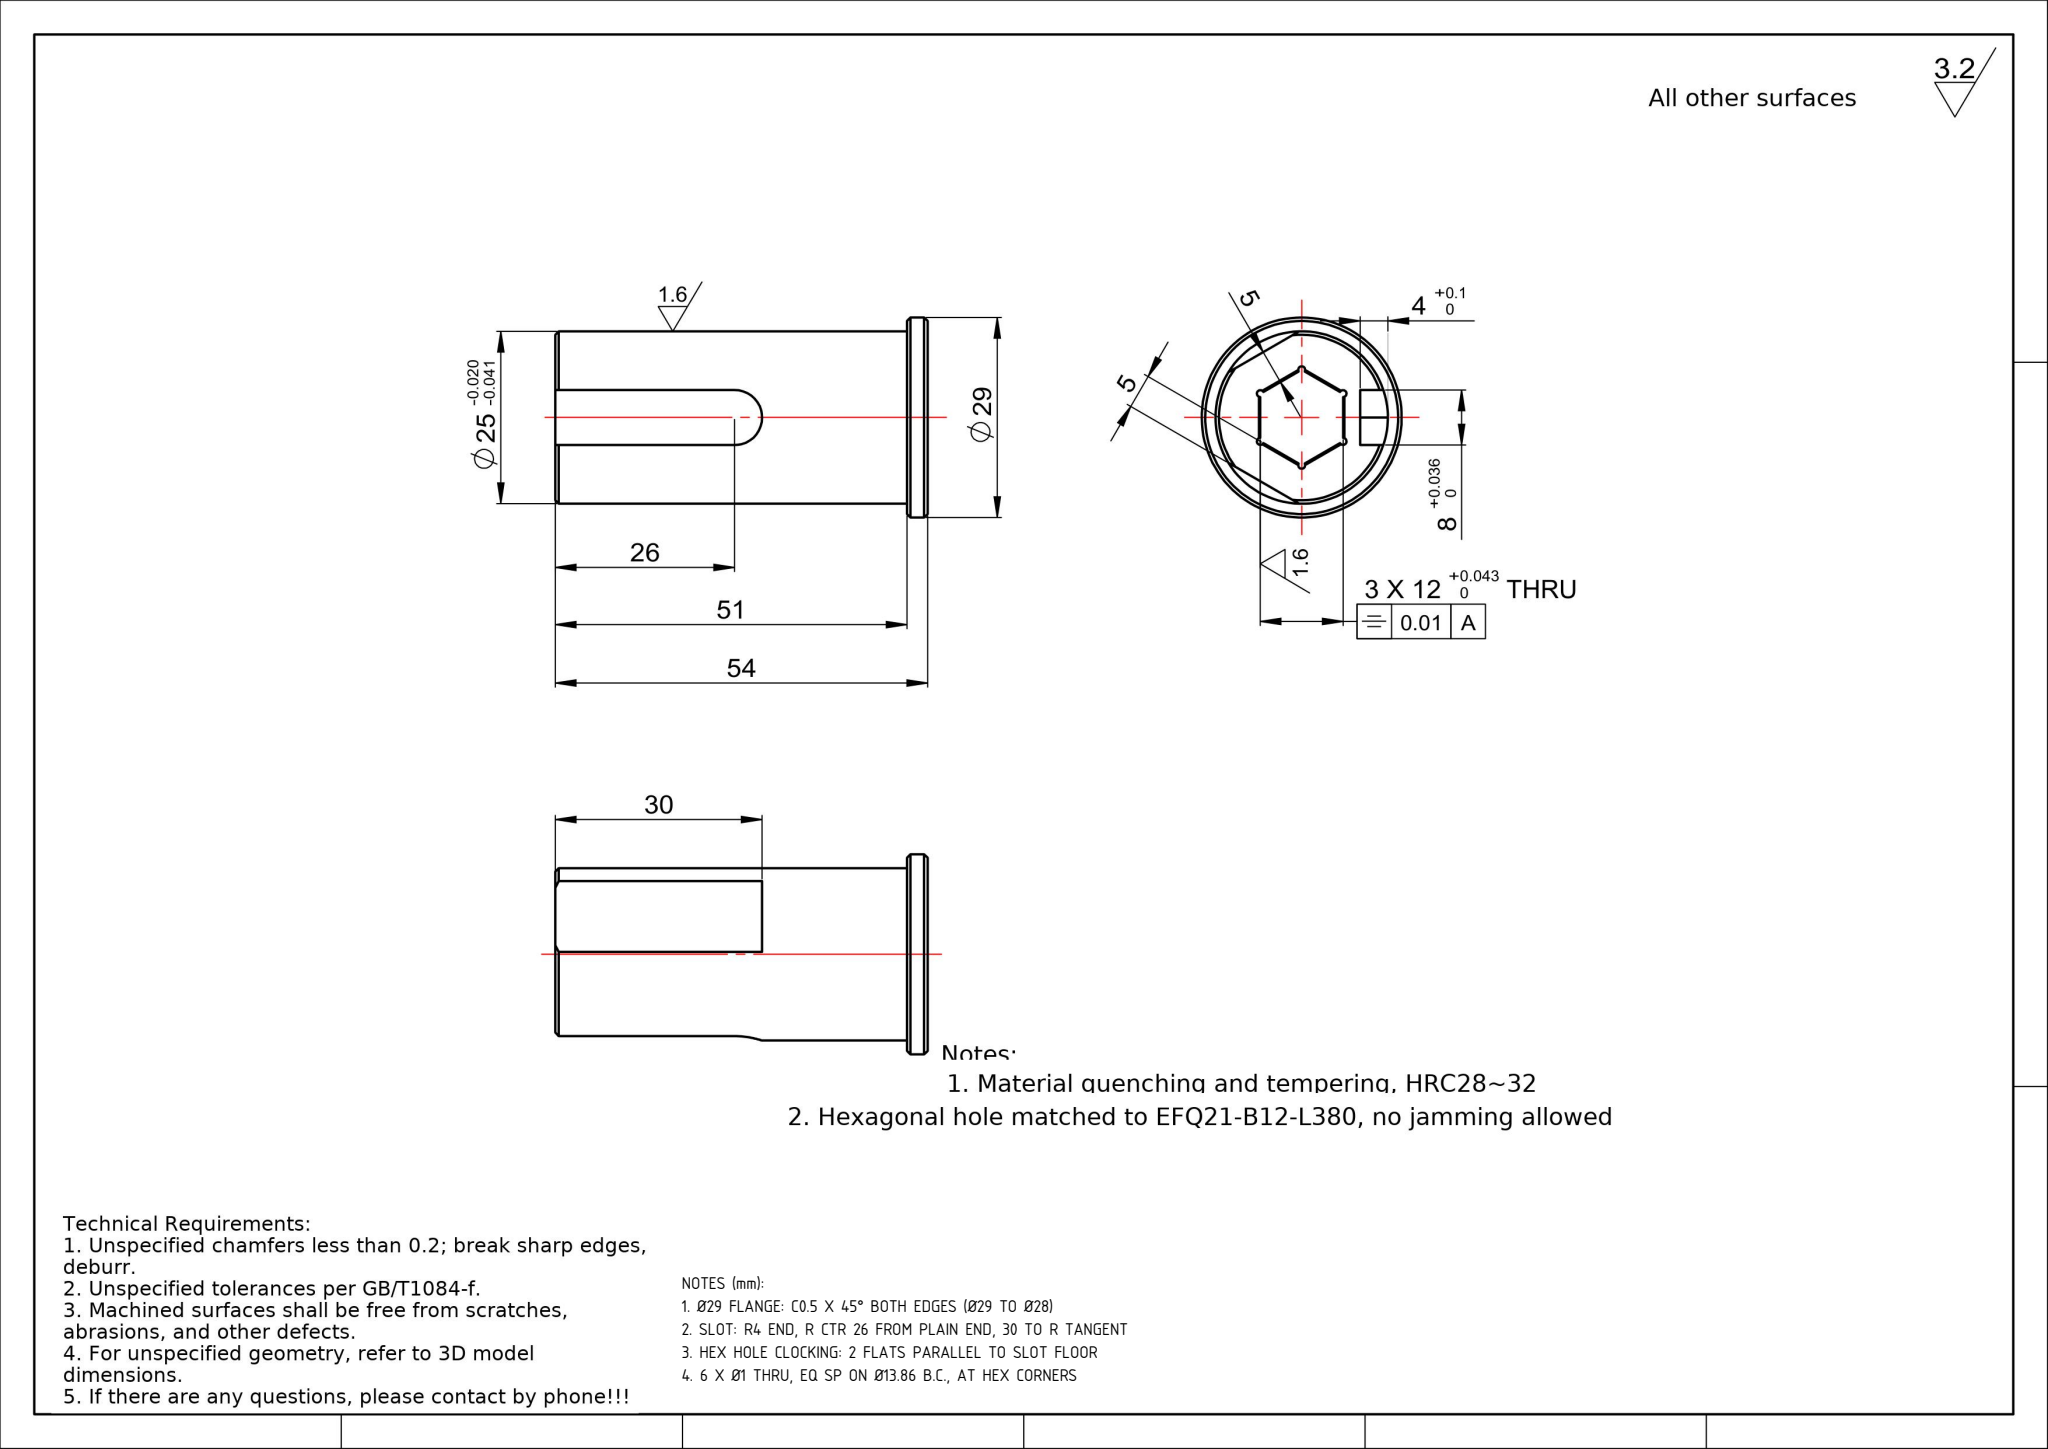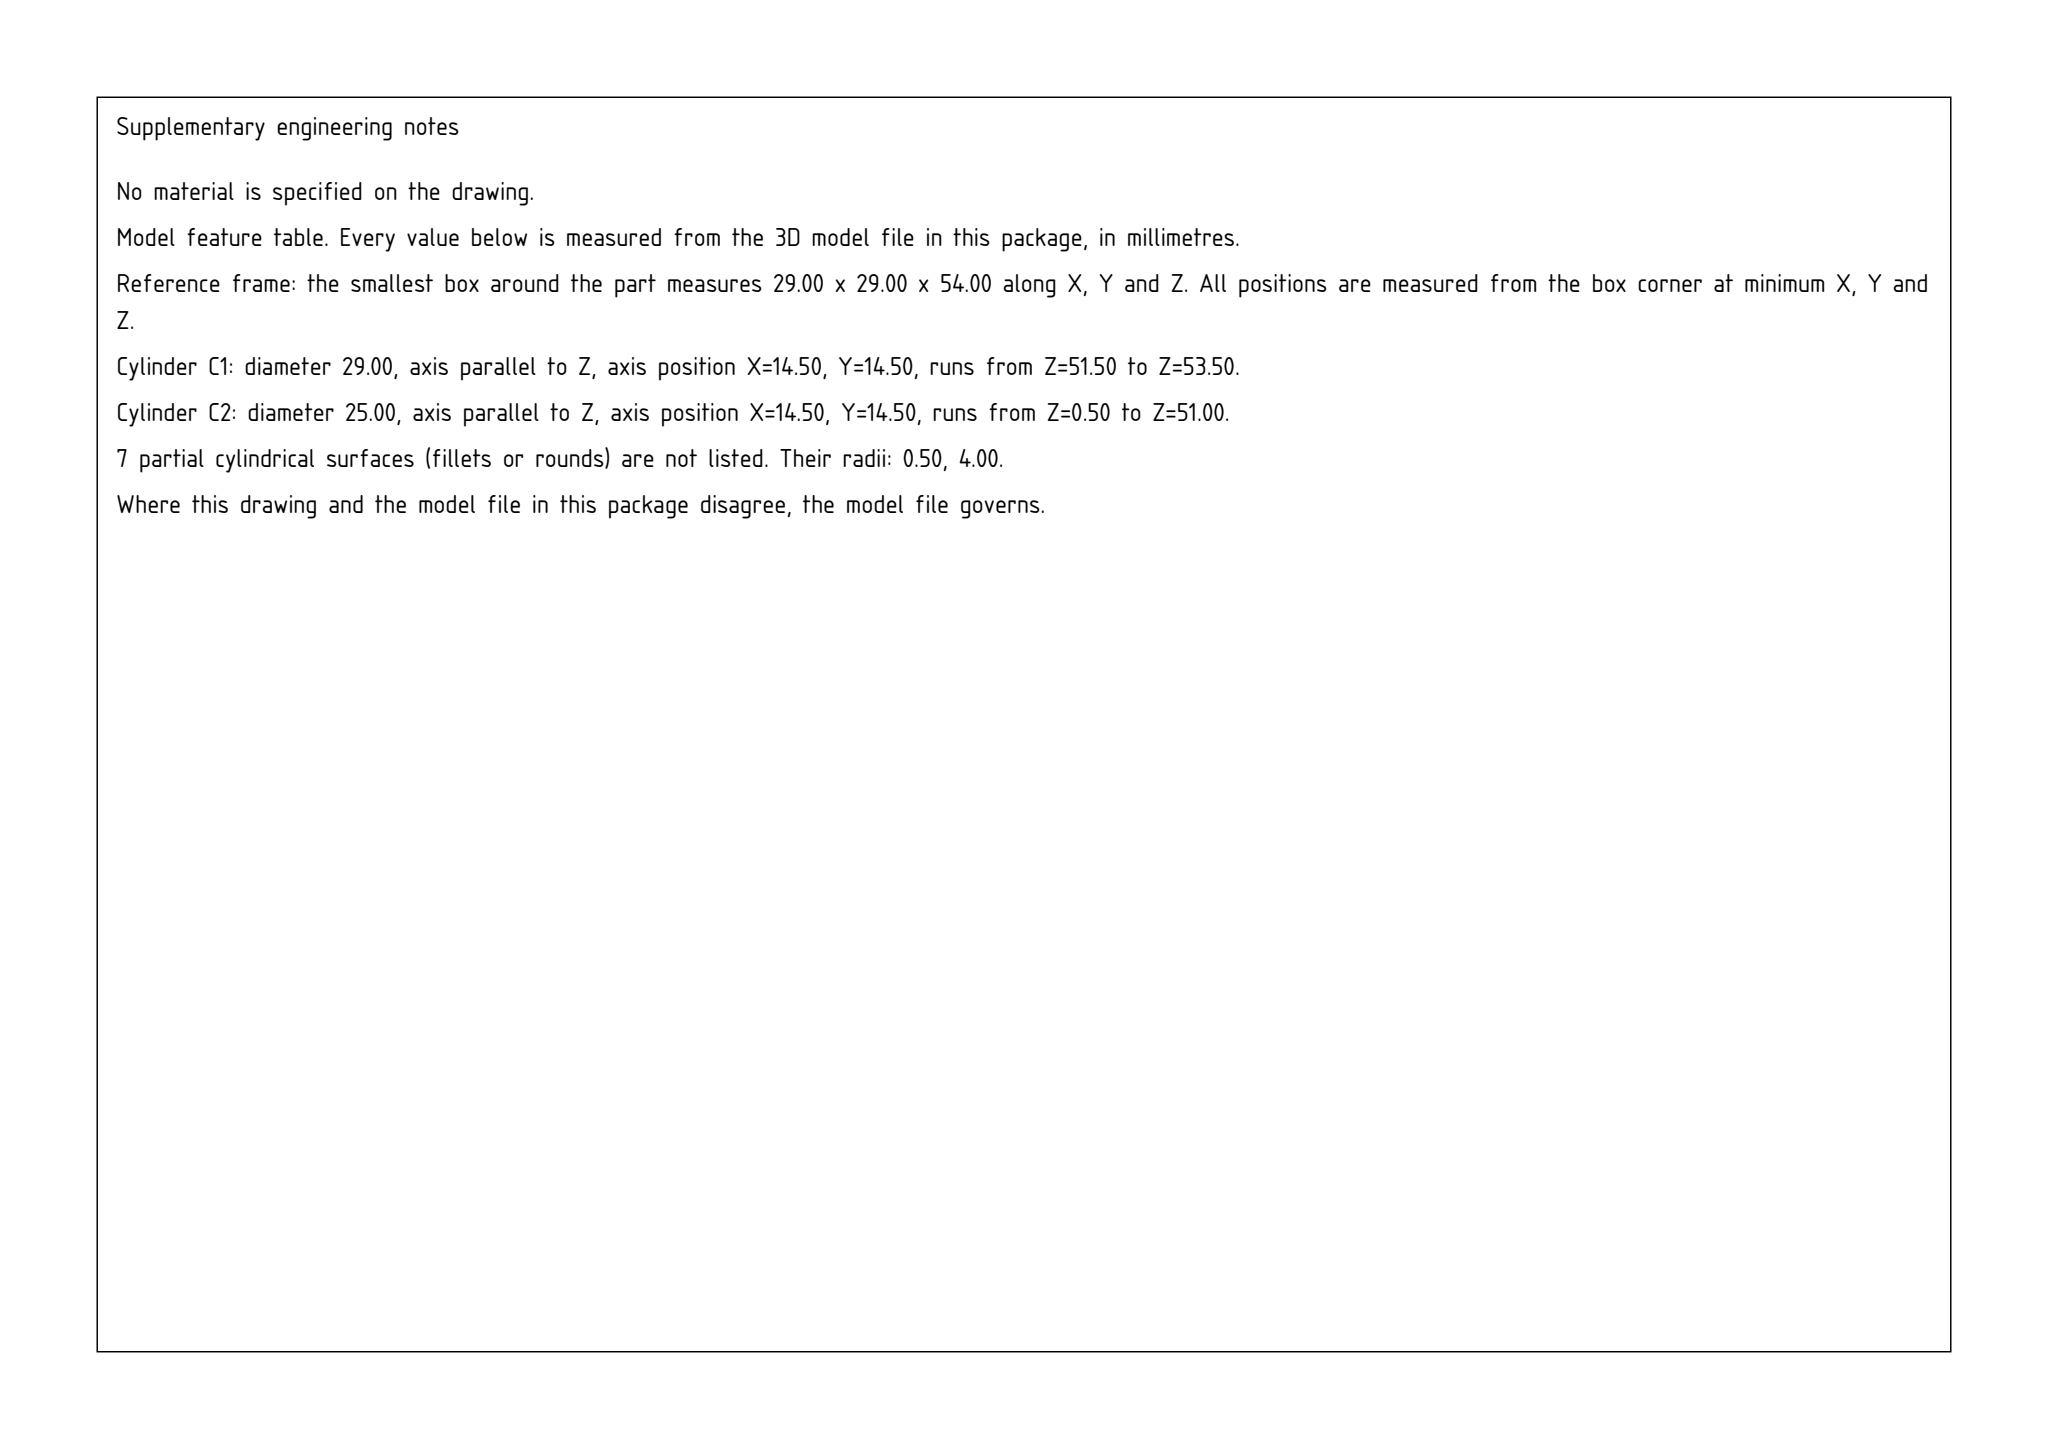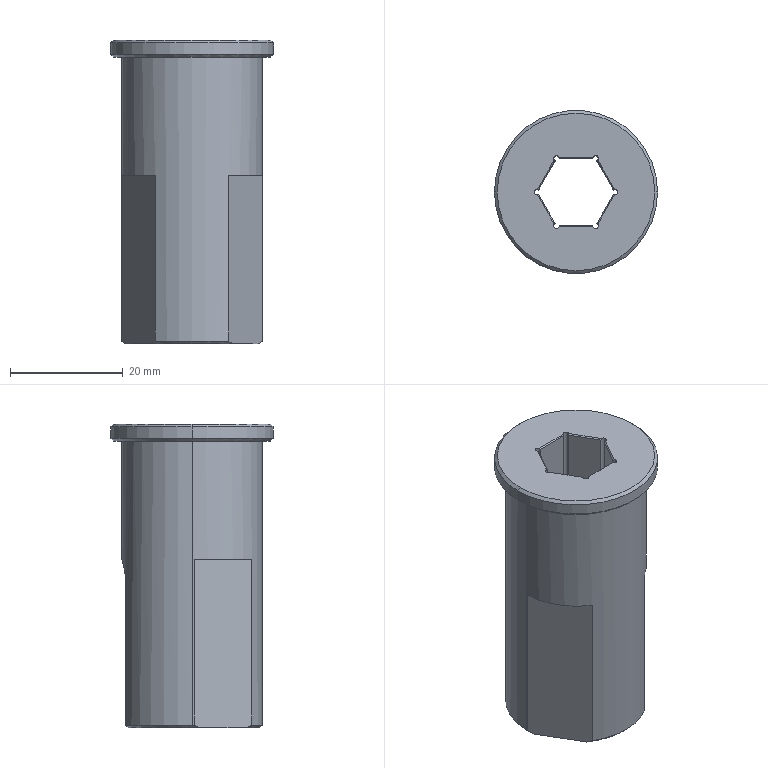Part | SolidWorks | mm | 1 solid | 51 faces | box 29 x 29 x 54 mm | volume 18478 mm3 | plane 28 | cylinder 15 | cone 8 | commonest cylinder face diameters 1 x9 29 x2 25 x2 8 x2
Drawing notes:
Ø29 FLANGE: C0.5 X 45° BOTH EDGES (Ø29 TO Ø28) | from the solid: Cones 90° incl, ref dia 29 (x2) and 28 (x2) on Ø29 flange, z=51-54
SLOT: R4 END, R CTR 26 FROM PLAIN END, 30 TO R TANGENT | from the solid: Ø8 cyl axis y at x14.5, z26, len 4 = R4 end; z-plane 30.0 = 26+4; x-planes 10.5/18.5, y-plane 23.0
HEX HOLE CLOCKING: 2 FLATS PARALLEL TO SLOT FLOOR | from the solid: Hex flat planes normal y at 8.5/20.5 (12 A/F) parallel to slot floor plane y=23
6 X Ø1 THRU, EQ SP ON Ø13.86 B.C., AT HEX CORNERS | from the solid: Six Ø1.0 z-axis cyls L=54 THRU at (7.57,14.5)(11.04,8.5)(11.04,20.5)(17.96,8.5)(17.96,20.5)(21.43,14.5), R6.93 from CL (14.5,14.5)